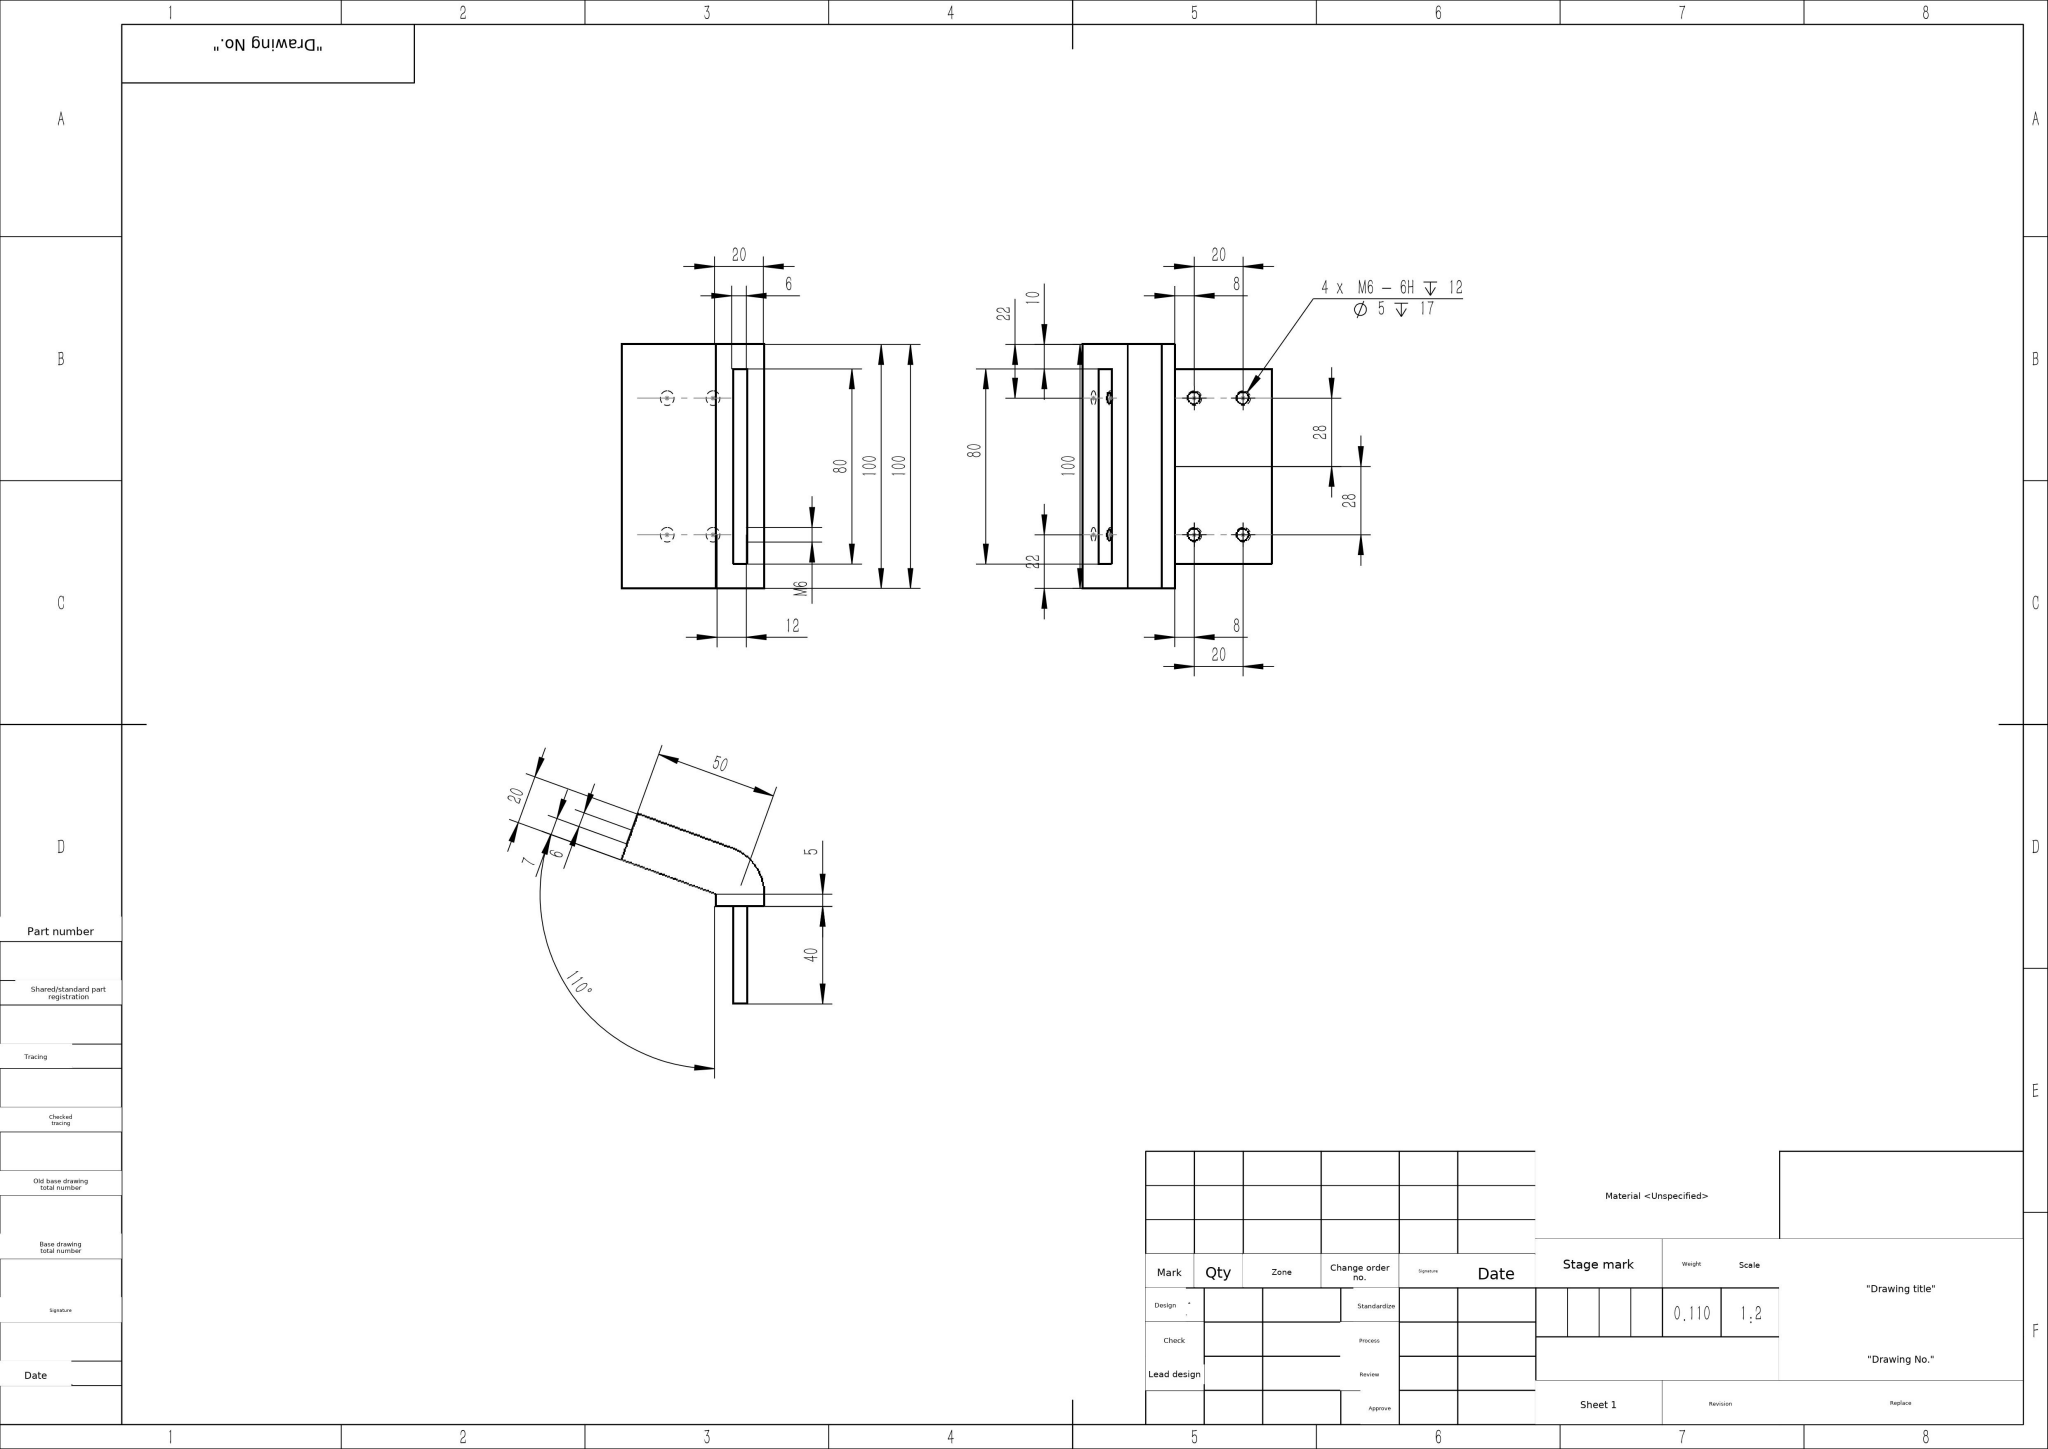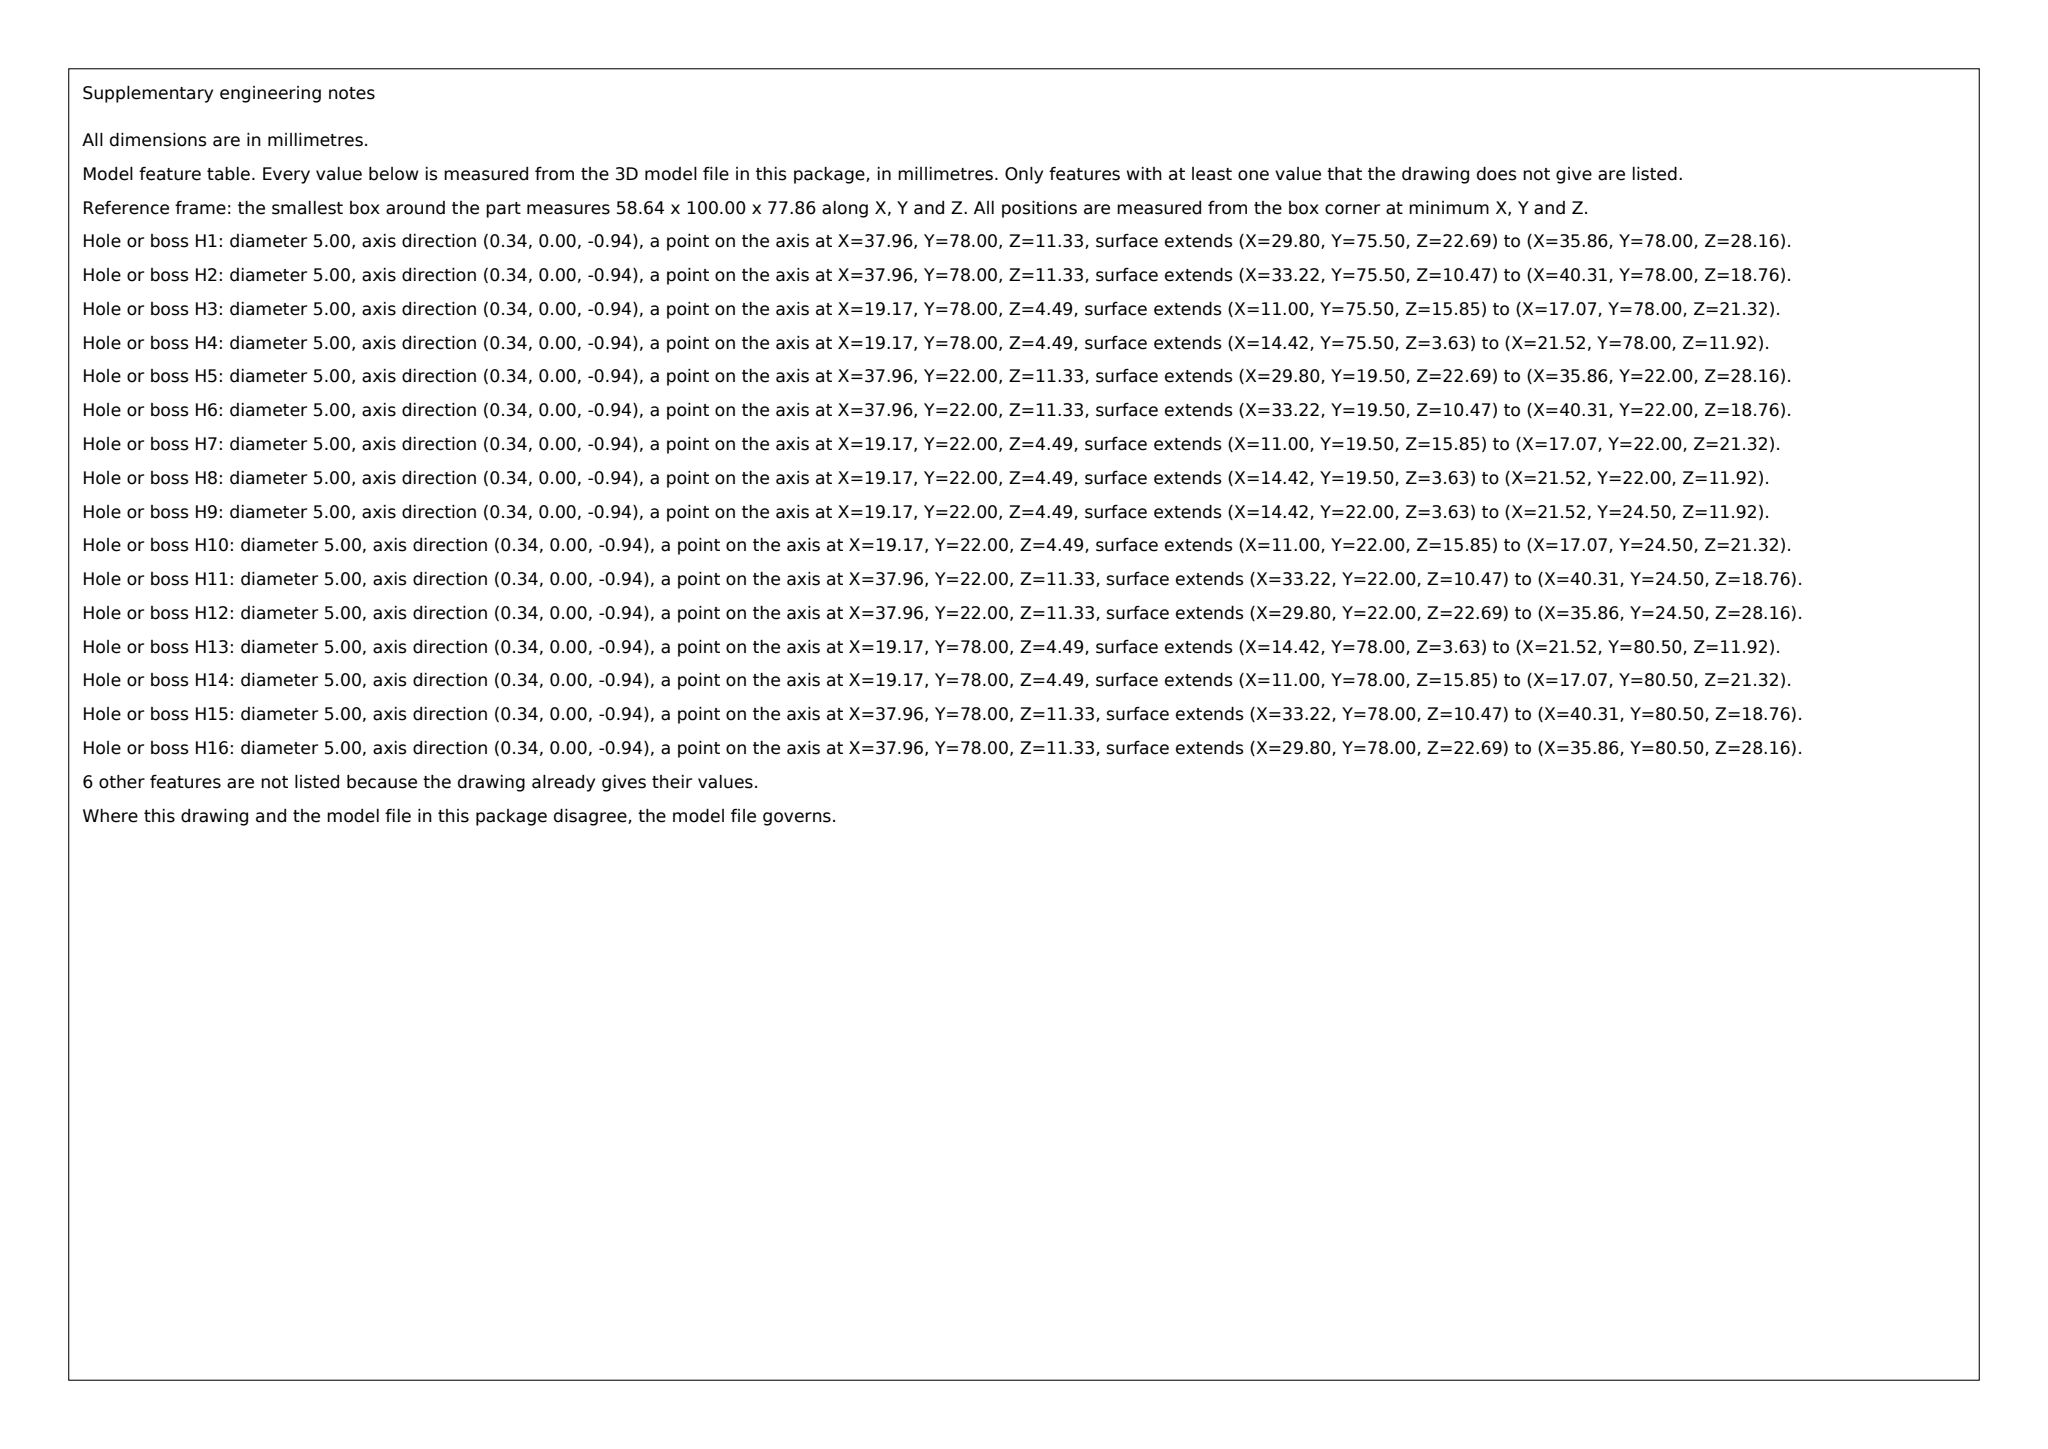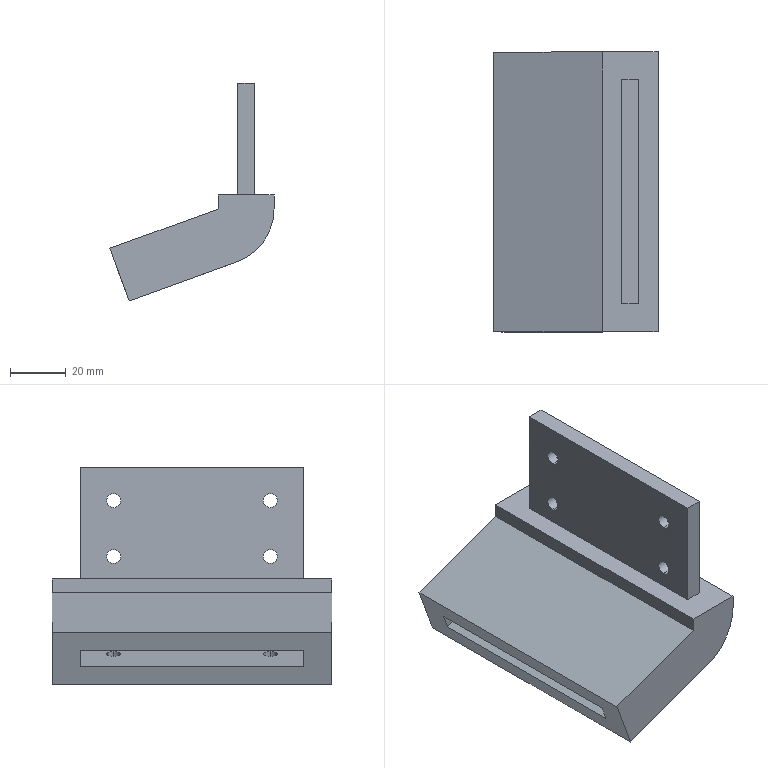Part | SolidWorks | mm | material <Unspecified> | 1 solid | 51 faces | box 58.64 x 100 x 77.86 mm | volume 110498 mm3 | cylinder 25 | plane 18 | cone 8 | commonest cylinder face diameters 5 x24 40 x1
build123d program:
from build123d import *

# Parameters (mm, degrees)
SKETCH1_W                       = 6
SKETCH1_H                       = 80
BOSS_EXTRUDE1_DEPTH             = 40
SKETCH5_W                       = 20
SKETCH5_H                       = 100
BOSS_EXTRUDE3_DEPTH             = 5
SKETCH8_W                       = 41.119
SKETCH8_H                       = 100
BOSS_EXTRUDE4_DEPTH             = 20
BOSS_EXTRUDE5_DEPTH             = 100
SKETCH10_W                      = 6
SKETCH10_H                      = 80
CUT_EXTRUDE1_DEPTH              = 50
M6_TAPPED_HOLE1_D               = 5
M6_TAPPED_HOLE1_DEPTH           = 17
M6_TAPPED_HOLE1_TIP             = 1.502
M6_TAPPED_HOLE2_D               = 5
M6_TAPPED_HOLE2_DEPTH           = 17
M6_TAPPED_HOLE2_TIP             = 1.502
M6_TAPPED_HOLE2_ON_FACE_2_D     = 5
M6_TAPPED_HOLE2_ON_FACE_2_DEPTH = 17
M6_TAPPED_HOLE2_ON_FACE_2_TIP   = 1.502
M6_TAPPED_HOLE2_ON_FACE_3_D     = 5
M6_TAPPED_HOLE2_ON_FACE_3_DEPTH = 17
M6_TAPPED_HOLE2_ON_FACE_3_TIP   = 1.502


with BuildPart() as part:
    # Sketch1 → Boss-Extrude1 (new body)
    with BuildSketch(Plane.XY):
        Rectangle(SKETCH1_W, SKETCH1_H)
    extrude(amount=BOSS_EXTRUDE1_DEPTH)

    # Sketch5 → Boss-Extrude3 (add)
    with BuildSketch(Plane(origin=(0, 0, 0), x_dir=(-1, 0, 0), z_dir=(0, 0, -1))):
        Rectangle(SKETCH5_W, SKETCH5_H)
    extrude(amount=BOSS_EXTRUDE3_DEPTH)



with BuildPart() as body_2:
    # Sketch8 → Boss-Extrude4 (new body)
    with BuildSketch(Plane(origin=(0.4372, 0, -1.201), x_dir=(-0.9397, 0, -0.342), z_dir=(-0.342, 0, 0.9397))):
        with Locations((31.666, 0)):
            Rectangle(SKETCH8_W, SKETCH8_H)
    extrude(amount=-BOSS_EXTRUDE4_DEPTH)


with BuildPart() as part_1:
    add(part.part)

    add(body_2.part)  # Boss-Extrude5 merges body 2
    # Sketch9 → Boss-Extrude5 (add)
    with BuildSketch(Plane.XZ.offset(50)):
        with BuildLine():
            Line((-10, -5), (10, -5))
            ThreePointArc((10, -5), (6.383, -16.472), (-3.16, -23.794))
            Line((-3.16, -23.794), (-10, -5))
        make_face()
    extrude(amount=-BOSS_EXTRUDE5_DEPTH)

    # Sketch10 → Cut-Extrude1 (cut)
    with BuildSketch(Plane(origin=(-49.076, 0, -17.862), x_dir=(-0.342, 0, 0.9397), z_dir=(-0.9397, 0, -0.342))):
        with Locations((-11.278, 0)):
            Rectangle(SKETCH10_W, SKETCH10_H)
    extrude(amount=-CUT_EXTRUDE1_DEPTH, mode=Mode.SUBTRACT)

    # M6 Tapped Hole1
    with Locations(Plane(origin=(3, 0, 0), x_dir=(0, 0, -1), z_dir=(1, 0, 0))):
        with Locations((-28, 28), (-8, 28), (-8, -28), (-28, -28)):
            Hole(M6_TAPPED_HOLE1_D / 2, depth=M6_TAPPED_HOLE1_DEPTH)
            with Locations((0, 0, -(M6_TAPPED_HOLE1_DEPTH + M6_TAPPED_HOLE1_TIP / 2))):  # 118° drill point
                Cone(0, M6_TAPPED_HOLE1_D / 2, M6_TAPPED_HOLE1_TIP, mode=Mode.SUBTRACT)

    # M6 Tapped Hole2
    with Locations(Plane(origin=(-10.677, 28, -26.53), x_dir=(-0.9397, 0, -0.342), z_dir=(0.342, 0, -0.9397))):
        with Locations((0, 0)):
            Hole(M6_TAPPED_HOLE2_D / 2, depth=M6_TAPPED_HOLE2_DEPTH)
            with Locations((0, 0, -(M6_TAPPED_HOLE2_DEPTH + M6_TAPPED_HOLE2_TIP / 2))):  # 118° drill point
                Cone(0, M6_TAPPED_HOLE2_D / 2, M6_TAPPED_HOLE2_TIP, mode=Mode.SUBTRACT)

    # M6 Tapped Hole2 on face 2
    with Locations(Plane(origin=(-29.471, 28, -33.37), x_dir=(-0.9397, 0, -0.342), z_dir=(0.342, 0, -0.9397))):
        with Locations((0, 0), (0, -56)):
            Hole(M6_TAPPED_HOLE2_ON_FACE_2_D / 2, depth=M6_TAPPED_HOLE2_ON_FACE_2_DEPTH)
            with Locations((0, 0, -(M6_TAPPED_HOLE2_ON_FACE_2_DEPTH + M6_TAPPED_HOLE2_ON_FACE_2_TIP / 2))):  # 118° drill point
                Cone(0, M6_TAPPED_HOLE2_ON_FACE_2_D / 2, M6_TAPPED_HOLE2_ON_FACE_2_TIP, mode=Mode.SUBTRACT)

    # M6 Tapped Hole2 on face 3
    with Locations(Plane(origin=(-10.677, -28, -26.53), x_dir=(-0.9397, 0, -0.342), z_dir=(0.342, 0, -0.9397))):
        with Locations((0, 0)):
            Hole(M6_TAPPED_HOLE2_ON_FACE_3_D / 2, depth=M6_TAPPED_HOLE2_ON_FACE_3_DEPTH)
            with Locations((0, 0, -(M6_TAPPED_HOLE2_ON_FACE_3_DEPTH + M6_TAPPED_HOLE2_ON_FACE_3_TIP / 2))):  # 118° drill point
                Cone(0, M6_TAPPED_HOLE2_ON_FACE_3_D / 2, M6_TAPPED_HOLE2_ON_FACE_3_TIP, mode=Mode.SUBTRACT)


solid = part_1.part